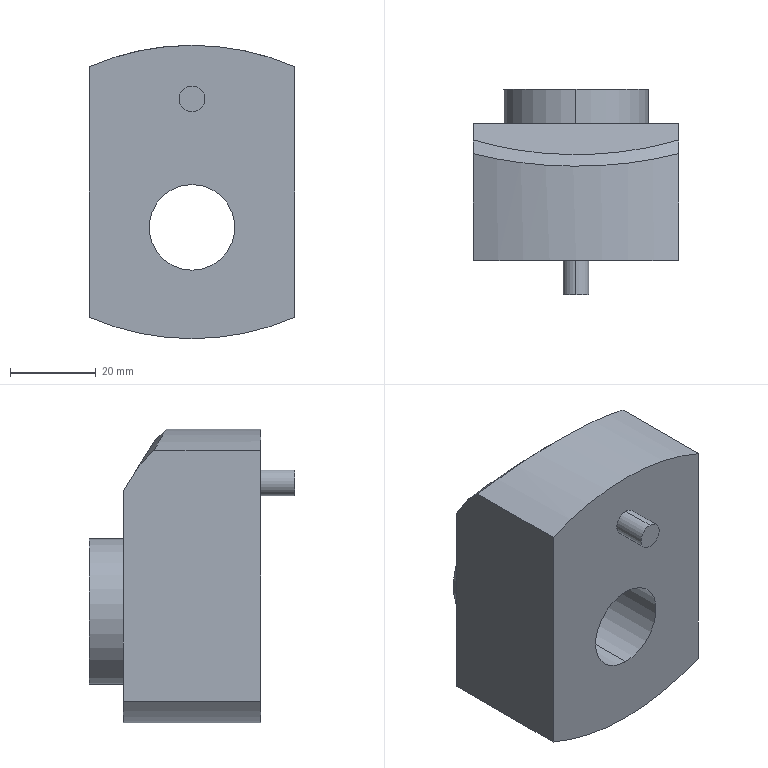Component | SolidWorks | DigitalDisplay.0-1 | 1 solid | 17 faces | box 48 x 48 x 68.5 mm | volume 92589 mm3 | cylinder 9 | plane 7 | spline 1 | commonest cylinder face diameters 120.2 x3 6 x2 20 x2 34 x2
STEP:
#1=COLOUR_RGB('',0.7922,0.8196,0.9333);
#2=FILL_AREA_STYLE_COLOUR('',#1);
#3=FILL_AREA_STYLE('',(#2));
#4=SURFACE_STYLE_FILL_AREA(#3);
#5=SURFACE_SIDE_STYLE('',(#4));
#6=SURFACE_STYLE_USAGE(.BOTH.,#5);
#7=PRESENTATION_STYLE_ASSIGNMENT((#6));
#8=CARTESIAN_POINT('',(-1.162,10.299,19.094));
#9=VERTEX_POINT('',#8);
#10=CARTESIAN_POINT('',(-1.162,10.299,19.331));
#11=VERTEX_POINT('',#10);
#12=CARTESIAN_POINT('',(-1.162,10.299,19.213));
#13=DIRECTION('',(0.,-1.,0.));
#14=DIRECTION('',(0.,0.,-1.));
#15=AXIS2_PLACEMENT_3D('',#12,#13,#14);
#16=CIRCLE('',#15,0.1181);
#17=EDGE_CURVE('',#9,#11,#16,.T.);
#18=ORIENTED_EDGE('',*,*,#17,.F.);
#19=CARTESIAN_POINT('',(-1.162,10.614,19.094));
#20=VERTEX_POINT('',#19);
#21=CARTESIAN_POINT('',(-1.162,10.299,19.094));
#22=DIRECTION('',(0.,1.,0.));
#23=VECTOR('',#22,39.37);
#24=LINE('',#21,#23);
#25=EDGE_CURVE('',#9,#20,#24,.T.);
#26=ORIENTED_EDGE('',*,*,#25,.T.);
#27=CARTESIAN_POINT('',(-1.162,10.614,19.331));
#28=VERTEX_POINT('',#27);
#29=CARTESIAN_POINT('',(-1.162,10.614,19.213));
#30=DIRECTION('',(0.,-1.,0.));
#31=DIRECTION('',(0.,0.,-1.));
#32=AXIS2_PLACEMENT_3D('',#29,#30,#31);
#33=CIRCLE('',#32,0.1181);
#34=EDGE_CURVE('',#20,#28,#33,.T.);
#35=ORIENTED_EDGE('',*,*,#34,.T.);
#36=CARTESIAN_POINT('',(-1.162,10.299,19.331));
#37=DIRECTION('',(0.,1.,0.));
#38=VECTOR('',#37,39.37);
#39=LINE('',#36,#38);
#40=EDGE_CURVE('',#11,#28,#39,.T.);
#41=ORIENTED_EDGE('',*,*,#40,.F.);
#42=EDGE_LOOP('',(#18,#26,#35,#41));
#43=FACE_OUTER_BOUND('',#42,.T.);
#44=CARTESIAN_POINT('',(-1.162,10.299,19.213));
#45=DIRECTION('',(0.,1.,0.));
#46=DIRECTION('',(0.,0.,1.));
#47=AXIS2_PLACEMENT_3D('',#44,#45,#46);
#48=CYLINDRICAL_SURFACE('',#47,0.1181);
#49=ADVANCED_FACE('',(#43),#48,.T.);
#50=CARTESIAN_POINT('',(-1.162,10.614,17.638));
#51=VERTEX_POINT('',#50);
#52=CARTESIAN_POINT('',(-1.162,10.614,18.425));
#53=VERTEX_POINT('',#52);
#54=CARTESIAN_POINT('',(-1.162,10.614,18.031));
#55=DIRECTION('',(0.,1.,0.));
#56=DIRECTION('',(0.,0.,1.));
#57=AXIS2_PLACEMENT_3D('',#54,#55,#56);
#58=CIRCLE('',#57,0.3937);
#59=EDGE_CURVE('',#51,#53,#58,.T.);
#60=ORIENTED_EDGE('',*,*,#59,.F.);
#61=CARTESIAN_POINT('',(-1.162,12.189,17.638));
#62=VERTEX_POINT('',#61);
#63=CARTESIAN_POINT('',(-1.162,10.614,17.638));
#64=DIRECTION('',(0.,1.,0.));
#65=VECTOR('',#64,39.37);
#66=LINE('',#63,#65);
#67=EDGE_CURVE('',#51,#62,#66,.T.);
#68=ORIENTED_EDGE('',*,*,#67,.T.);
#69=CARTESIAN_POINT('',(-1.162,12.189,18.425));
#70=VERTEX_POINT('',#69);
#71=CARTESIAN_POINT('',(-1.162,12.189,18.031));
#72=DIRECTION('',(0.,1.,0.));
#73=DIRECTION('',(0.,0.,1.));
#74=AXIS2_PLACEMENT_3D('',#71,#72,#73);
#75=CIRCLE('',#74,0.3937);
#76=EDGE_CURVE('',#62,#70,#75,.T.);
#77=ORIENTED_EDGE('',*,*,#76,.T.);
#78=CARTESIAN_POINT('',(-1.162,10.614,18.425));
#79=DIRECTION('',(0.,1.,0.));
#80=VECTOR('',#79,39.37);
#81=LINE('',#78,#80);
#82=EDGE_CURVE('',#53,#70,#81,.T.);
#83=ORIENTED_EDGE('',*,*,#82,.F.);
#84=EDGE_LOOP('',(#60,#68,#77,#83));
#85=FACE_OUTER_BOUND('',#84,.T.);
#86=CARTESIAN_POINT('',(-1.162,10.614,18.031));
#87=DIRECTION('',(0.,1.,0.));
#88=DIRECTION('',(0.,0.,1.));
#89=AXIS2_PLACEMENT_3D('',#86,#87,#88);
#90=CYLINDRICAL_SURFACE('',#89,0.3937);
#91=ADVANCED_FACE('',(#85),#90,.F.);
#92=CARTESIAN_POINT('',(-1.162,12.189,18.701));
#93=VERTEX_POINT('',#92);
#94=CARTESIAN_POINT('',(-1.162,12.189,17.362));
#95=VERTEX_POINT('',#94);
#96=CARTESIAN_POINT('',(-1.162,12.189,18.031));
#97=DIRECTION('',(0.,1.,0.));
#98=DIRECTION('',(0.,0.,1.));
#99=AXIS2_PLACEMENT_3D('',#96,#97,#98);
#100=CIRCLE('',#99,0.6693);
#101=EDGE_CURVE('',#93,#95,#100,.T.);
#102=ORIENTED_EDGE('',*,*,#101,.F.);
#103=CARTESIAN_POINT('',(-1.162,11.874,18.701));
#104=VERTEX_POINT('',#103);
#105=CARTESIAN_POINT('',(-1.162,12.189,18.701));
#106=DIRECTION('',(0.,-1.,0.));
#107=VECTOR('',#106,39.37);
#108=LINE('',#105,#107);
#109=EDGE_CURVE('',#93,#104,#108,.T.);
#110=ORIENTED_EDGE('',*,*,#109,.T.);
#111=CARTESIAN_POINT('',(-1.162,11.874,17.362));
#112=VERTEX_POINT('',#111);
#113=CARTESIAN_POINT('',(-1.162,11.874,18.031));
#114=DIRECTION('',(0.,1.,0.));
#115=DIRECTION('',(0.,0.,-1.));
#116=AXIS2_PLACEMENT_3D('',#113,#114,#115);
#117=CIRCLE('',#116,0.6693);
#118=EDGE_CURVE('',#104,#112,#117,.T.);
#119=ORIENTED_EDGE('',*,*,#118,.T.);
#120=CARTESIAN_POINT('',(-1.162,12.189,17.362));
#121=DIRECTION('',(0.,-1.,0.));
#122=VECTOR('',#121,39.37);
#123=LINE('',#120,#122);
#124=EDGE_CURVE('',#95,#112,#123,.T.);
#125=ORIENTED_EDGE('',*,*,#124,.F.);
#126=EDGE_LOOP('',(#102,#110,#119,#125));
#127=FACE_OUTER_BOUND('',#126,.T.);
#128=CARTESIAN_POINT('',(-1.162,12.189,18.031));
#129=DIRECTION('',(0.,-1.,0.));
#130=DIRECTION('',(0.,0.,-1.));
#131=AXIS2_PLACEMENT_3D('',#128,#129,#130);
#132=CYLINDRICAL_SURFACE('',#131,0.6693);
#133=ADVANCED_FACE('',(#127),#132,.T.);
#134=CARTESIAN_POINT('',(-1.162,11.874,17.008));
#135=VERTEX_POINT('',#134);
#136=CARTESIAN_POINT('',(-2.107,11.874,17.205));
#137=VERTEX_POINT('',#136);
#138=CARTESIAN_POINT('',(-1.162,11.874,19.374));
#139=DIRECTION('',(0.,1.,0.));
#140=DIRECTION('',(0.,0.,-1.));
#141=AXIS2_PLACEMENT_3D('',#138,#139,#140);
#142=CIRCLE('',#141,2.366);
#143=EDGE_CURVE('',#135,#137,#142,.T.);
#144=ORIENTED_EDGE('',*,*,#143,.F.);
#145=CARTESIAN_POINT('',(-1.162,10.614,17.008));
#146=VERTEX_POINT('',#145);
#147=CARTESIAN_POINT('',(-1.162,11.874,17.008));
#148=DIRECTION('',(0.,-1.,0.));
#149=VECTOR('',#148,39.37);
#150=LINE('',#147,#149);
#151=EDGE_CURVE('',#135,#146,#150,.T.);
#152=ORIENTED_EDGE('',*,*,#151,.T.);
#153=CARTESIAN_POINT('',(-2.107,10.614,17.205));
#154=VERTEX_POINT('',#153);
#155=CARTESIAN_POINT('',(-1.162,10.614,19.374));
#156=DIRECTION('',(0.,1.,0.));
#157=DIRECTION('',(0.,0.,-1.));
#158=AXIS2_PLACEMENT_3D('',#155,#156,#157);
#159=CIRCLE('',#158,2.366);
#160=EDGE_CURVE('',#146,#154,#159,.T.);
#161=ORIENTED_EDGE('',*,*,#160,.T.);
#162=CARTESIAN_POINT('',(-2.107,11.874,17.205));
#163=DIRECTION('',(0.,-1.,0.));
#164=VECTOR('',#163,39.37);
#165=LINE('',#162,#164);
#166=EDGE_CURVE('',#137,#154,#165,.T.);
#167=ORIENTED_EDGE('',*,*,#166,.F.);
#168=EDGE_LOOP('',(#144,#152,#161,#167));
#169=FACE_OUTER_BOUND('',#168,.T.);
#170=CARTESIAN_POINT('',(-1.162,11.874,19.374));
#171=DIRECTION('',(0.,-1.,0.));
#172=DIRECTION('',(0.,0.,-1.));
#173=AXIS2_PLACEMENT_3D('',#170,#171,#172);
#174=CYLINDRICAL_SURFACE('',#173,2.366);
#175=ADVANCED_FACE('',(#169),#174,.T.);
#176=CARTESIAN_POINT('',(-2.107,11.595,19.508));
#177=VERTEX_POINT('',#176);
#178=CARTESIAN_POINT('',(-2.107,10.614,19.508));
#179=VERTEX_POINT('',#178);
#180=CARTESIAN_POINT('',(-2.107,11.874,19.508));
#181=DIRECTION('',(0.,-1.,0.));
#182=VECTOR('',#181,39.37);
#183=LINE('',#180,#182);
#184=EDGE_CURVE('',#177,#179,#183,.T.);
#185=ORIENTED_EDGE('',*,*,#184,.F.);
#186=CARTESIAN_POINT('',(-2.107,11.722,19.384));
#187=VERTEX_POINT('',#186);
#188=CARTESIAN_POINT('',(-2.107,11.595,19.508));
#189=CARTESIAN_POINT('',(-2.107,11.64,19.464));
#190=CARTESIAN_POINT('',(-2.107,11.682,19.423));
#191=CARTESIAN_POINT('',(-2.107,11.722,19.384));
#192=B_SPLINE_CURVE_WITH_KNOTS('',3,(#188,#189,#190,#191),.UNSPECIFIED.,.F.,.F.,(4,4),(0.,1.),.UNSPECIFIED.);
#193=EDGE_CURVE('',#177,#187,#192,.T.);
#194=ORIENTED_EDGE('',*,*,#193,.T.);
#195=CARTESIAN_POINT('',(-2.107,11.874,19.144));
#196=VERTEX_POINT('',#195);
#197=CARTESIAN_POINT('',(-2.107,12.749,17.758));
#198=DIRECTION('',(0.,-0.534,0.8455));
#199=VECTOR('',#198,39.37);
#200=LINE('',#197,#199);
#201=EDGE_CURVE('',#196,#187,#200,.T.);
#202=ORIENTED_EDGE('',*,*,#201,.F.);
#203=CARTESIAN_POINT('',(-2.107,11.874,17.205));
#204=DIRECTION('',(0.,0.,1.));
#205=VECTOR('',#204,39.37);
#206=LINE('',#203,#205);
#207=EDGE_CURVE('',#137,#196,#206,.T.);
#208=ORIENTED_EDGE('',*,*,#207,.F.);
#209=ORIENTED_EDGE('',*,*,#166,.T.);
#210=CARTESIAN_POINT('',(-2.107,10.614,17.205));
#211=DIRECTION('',(0.,0.,1.));
#212=VECTOR('',#211,39.37);
#213=LINE('',#210,#212);
#214=EDGE_CURVE('',#154,#179,#213,.T.);
#215=ORIENTED_EDGE('',*,*,#214,.T.);
#216=EDGE_LOOP('',(#185,#194,#202,#208,#209,#215));
#217=FACE_OUTER_BOUND('',#216,.T.);
#218=CARTESIAN_POINT('',(-2.107,11.874,17.205));
#219=DIRECTION('',(1.,0.,-0.));
#220=DIRECTION('',(-0.,0.,-1.));
#221=AXIS2_PLACEMENT_3D('',#218,#219,#220);
#222=PLANE('',#221);
#223=ADVANCED_FACE('',(#217),#222,.F.);
#224=CARTESIAN_POINT('',(-0.2168,11.595,19.508));
#225=VERTEX_POINT('',#224);
#226=CARTESIAN_POINT('',(-0.2168,10.614,19.508));
#227=VERTEX_POINT('',#226);
#228=CARTESIAN_POINT('',(-0.2168,11.874,19.508));
#229=DIRECTION('',(0.,-1.,0.));
#230=VECTOR('',#229,39.37);
#231=LINE('',#228,#230);
#232=EDGE_CURVE('',#225,#227,#231,.T.);
#233=ORIENTED_EDGE('',*,*,#232,.F.);
#234=CARTESIAN_POINT('',(-0.2168,11.595,19.508));
#235=CARTESIAN_POINT('',(-0.2542,11.586,19.524));
#236=CARTESIAN_POINT('',(-0.2918,11.577,19.539));
#237=CARTESIAN_POINT('',(-0.3487,11.564,19.561));
#238=CARTESIAN_POINT('',(-0.3772,11.558,19.571));
#239=CARTESIAN_POINT('',(-0.4106,11.551,19.582));
#240=CARTESIAN_POINT('',(-0.425,11.549,19.587));
#241=CARTESIAN_POINT('',(-0.4346,11.547,19.59));
#242=CARTESIAN_POINT('',(-0.4393,11.546,19.592));
#243=CARTESIAN_POINT('',(-0.4829,11.538,19.606));
#244=CARTESIAN_POINT('',(-0.5219,11.531,19.617));
#245=CARTESIAN_POINT('',(-0.5807,11.522,19.632));
#246=CARTESIAN_POINT('',(-0.6101,11.518,19.64));
#247=CARTESIAN_POINT('',(-0.6397,11.514,19.646));
#248=CARTESIAN_POINT('',(-0.6594,11.511,19.651));
#249=CARTESIAN_POINT('',(-0.6691,11.51,19.653));
#250=CARTESIAN_POINT('',(-0.7189,11.504,19.663));
#251=CARTESIAN_POINT('',(-0.7588,11.5,19.671));
#252=CARTESIAN_POINT('',(-0.8188,11.494,19.68));
#253=CARTESIAN_POINT('',(-0.8388,11.493,19.683));
#254=CARTESIAN_POINT('',(-0.8789,11.49,19.688));
#255=CARTESIAN_POINT('',(-0.8989,11.488,19.69));
#256=CARTESIAN_POINT('',(-0.9998,11.482,19.701));
#257=CARTESIAN_POINT('',(-1.081,11.48,19.705));
#258=CARTESIAN_POINT('',(-1.202,11.48,19.705));
#259=CARTESIAN_POINT('',(-1.243,11.48,19.704));
#260=CARTESIAN_POINT('',(-1.303,11.482,19.701));
#261=CARTESIAN_POINT('',(-1.323,11.483,19.699));
#262=CARTESIAN_POINT('',(-1.364,11.485,19.696));
#263=CARTESIAN_POINT('',(-1.384,11.486,19.694));
#264=CARTESIAN_POINT('',(-1.444,11.49,19.688));
#265=CARTESIAN_POINT('',(-1.485,11.493,19.683));
#266=CARTESIAN_POINT('',(-1.545,11.498,19.674));
#267=CARTESIAN_POINT('',(-1.575,11.501,19.669));
#268=CARTESIAN_POINT('',(-1.604,11.504,19.663));
#269=CARTESIAN_POINT('',(-1.624,11.507,19.659));
#270=CARTESIAN_POINT('',(-1.634,11.508,19.657));
#271=CARTESIAN_POINT('',(-1.684,11.514,19.647));
#272=CARTESIAN_POINT('',(-1.723,11.519,19.638));
#273=CARTESIAN_POINT('',(-1.782,11.528,19.622));
#274=CARTESIAN_POINT('',(-1.811,11.533,19.614));
#275=CARTESIAN_POINT('',(-1.845,11.539,19.604));
#276=CARTESIAN_POINT('',(-1.86,11.541,19.599));
#277=CARTESIAN_POINT('',(-1.869,11.543,19.596));
#278=CARTESIAN_POINT('',(-1.874,11.544,19.595));
#279=CARTESIAN_POINT('',(-1.956,11.559,19.569));
#280=CARTESIAN_POINT('',(-2.032,11.576,19.54));
#281=CARTESIAN_POINT('',(-2.107,11.595,19.508));
#282=B_SPLINE_CURVE_WITH_KNOTS('',3,(#234,#235,#236,#237,#238,#239,#240,#241,#242,#243,#244,#245,#246,#247,#248,#249,#250,#251,#252,#253,#254,#255,#256,#257,#258,#259,#260,#261,#262,#263,#264,#265,#266,#267,#268,#269,#270,#271,#272,#273,#274,#275,#276,#277,#278,#279,#280,#281),.UNSPECIFIED.,.F.,.F.,(4,2,1,1,2,2,2,1,2,2,2,2,2,2,2,2,2,2,1,2,2,2,1,1,2,2,4),(0.,0.0625,0.09375,0.1094,0.1172,0.125,0.1875,0.2188,0.2344,0.25,0.3125,0.3438,0.375,0.5,0.5625,0.5938,0.625,0.6875,0.7188,0.7344,0.75,0.8125,0.8438,0.8594,0.8672,0.875,1.),.UNSPECIFIED.);
#283=EDGE_CURVE('',#225,#177,#282,.T.);
#284=ORIENTED_EDGE('',*,*,#283,.T.);
#285=ORIENTED_EDGE('',*,*,#184,.T.);
#286=CARTESIAN_POINT('',(-1.162,10.614,17.339));
#287=DIRECTION('',(0.,1.,0.));
#288=DIRECTION('',(0.,0.,-1.));
#289=AXIS2_PLACEMENT_3D('',#286,#287,#288);
#290=CIRCLE('',#289,2.366);
#291=EDGE_CURVE('',#179,#227,#290,.T.);
#292=ORIENTED_EDGE('',*,*,#291,.T.);
#293=EDGE_LOOP('',(#233,#284,#285,#292));
#294=FACE_OUTER_BOUND('',#293,.T.);
#295=CARTESIAN_POINT('',(-1.162,11.874,17.339));
#296=DIRECTION('',(0.,-1.,0.));
#297=DIRECTION('',(0.,0.,-1.));
#298=AXIS2_PLACEMENT_3D('',#295,#296,#297);
#299=CYLINDRICAL_SURFACE('',#298,2.366);
#300=ADVANCED_FACE('',(#294),#299,.T.);
#301=CARTESIAN_POINT('',(-0.2168,11.722,19.384));
#302=VERTEX_POINT('',#301);
#303=CARTESIAN_POINT('',(-0.2168,11.874,19.144));
#304=VERTEX_POINT('',#303);
#305=CARTESIAN_POINT('',(-0.2168,12.749,17.758));
#306=DIRECTION('',(-0.,0.534,-0.8455));
#307=VECTOR('',#306,39.37);
#308=LINE('',#305,#307);
#309=EDGE_CURVE('',#302,#304,#308,.T.);
#310=ORIENTED_EDGE('',*,*,#309,.F.);
#311=CARTESIAN_POINT('',(-0.2168,11.722,19.384));
#312=CARTESIAN_POINT('',(-0.2168,11.682,19.423));
#313=CARTESIAN_POINT('',(-0.2168,11.64,19.464));
#314=CARTESIAN_POINT('',(-0.2168,11.595,19.508));
#315=B_SPLINE_CURVE_WITH_KNOTS('',3,(#311,#312,#313,#314),.UNSPECIFIED.,.F.,.F.,(4,4),(0.,1.),.UNSPECIFIED.);
#316=EDGE_CURVE('',#302,#225,#315,.T.);
#317=ORIENTED_EDGE('',*,*,#316,.T.);
#318=ORIENTED_EDGE('',*,*,#232,.T.);
#319=CARTESIAN_POINT('',(-0.2168,10.614,17.205));
#320=VERTEX_POINT('',#319);
#321=CARTESIAN_POINT('',(-0.2168,10.614,17.205));
#322=DIRECTION('',(-0.,0.,-1.));
#323=VECTOR('',#322,39.37);
#324=LINE('',#321,#323);
#325=EDGE_CURVE('',#227,#320,#324,.T.);
#326=ORIENTED_EDGE('',*,*,#325,.T.);
#327=CARTESIAN_POINT('',(-0.2168,11.874,17.205));
#328=VERTEX_POINT('',#327);
#329=CARTESIAN_POINT('',(-0.2168,11.874,17.205));
#330=DIRECTION('',(0.,-1.,0.));
#331=VECTOR('',#330,39.37);
#332=LINE('',#329,#331);
#333=EDGE_CURVE('',#328,#320,#332,.T.);
#334=ORIENTED_EDGE('',*,*,#333,.F.);
#335=CARTESIAN_POINT('',(-0.2168,11.874,17.205));
#336=DIRECTION('',(-0.,0.,-1.));
#337=VECTOR('',#336,39.37);
#338=LINE('',#335,#337);
#339=EDGE_CURVE('',#304,#328,#338,.T.);
#340=ORIENTED_EDGE('',*,*,#339,.F.);
#341=EDGE_LOOP('',(#310,#317,#318,#326,#334,#340));
#342=FACE_OUTER_BOUND('',#341,.T.);
#343=CARTESIAN_POINT('',(-0.2168,11.874,17.205));
#344=DIRECTION('',(-1.,0.,0.));
#345=DIRECTION('',(0.,0.,1.));
#346=AXIS2_PLACEMENT_3D('',#343,#344,#345);
#347=PLANE('',#346);
#348=ADVANCED_FACE('',(#342),#347,.F.);
#349=CARTESIAN_POINT('',(-1.162,11.874,18.031));
#350=DIRECTION('',(0.,1.,0.));
#351=DIRECTION('',(0.,0.,-1.));
#352=AXIS2_PLACEMENT_3D('',#349,#350,#351);
#353=CIRCLE('',#352,0.6693);
#354=EDGE_CURVE('',#112,#104,#353,.T.);
#355=ORIENTED_EDGE('',*,*,#354,.F.);
#356=ORIENTED_EDGE('',*,*,#118,.F.);
#357=EDGE_LOOP('',(#355,#356));
#358=FACE_BOUND('',#357,.T.);
#359=CARTESIAN_POINT('',(-1.162,11.874,19.144));
#360=DIRECTION('',(-1.,0.,0.));
#361=VECTOR('',#360,39.37);
#362=LINE('',#359,#361);
#363=EDGE_CURVE('',#304,#196,#362,.T.);
#364=ORIENTED_EDGE('',*,*,#363,.F.);
#365=ORIENTED_EDGE('',*,*,#339,.T.);
#366=CARTESIAN_POINT('',(-1.162,11.874,19.374));
#367=DIRECTION('',(0.,1.,0.));
#368=DIRECTION('',(0.,0.,-1.));
#369=AXIS2_PLACEMENT_3D('',#366,#367,#368);
#370=CIRCLE('',#369,2.366);
#371=EDGE_CURVE('',#328,#135,#370,.T.);
#372=ORIENTED_EDGE('',*,*,#371,.T.);
#373=ORIENTED_EDGE('',*,*,#143,.T.);
#374=ORIENTED_EDGE('',*,*,#207,.T.);
#375=EDGE_LOOP('',(#364,#365,#372,#373,#374));
#376=FACE_OUTER_BOUND('',#375,.T.);
#377=CARTESIAN_POINT('',(-1.162,11.874,19.374));
#378=DIRECTION('',(0.,-1.,0.));
#379=DIRECTION('',(0.,0.,-1.));
#380=AXIS2_PLACEMENT_3D('',#377,#378,#379);
#381=PLANE('',#380);
#382=ADVANCED_FACE('',(#358,#376),#381,.F.);
#383=ORIENTED_EDGE('',*,*,#151,.F.);
#384=ORIENTED_EDGE('',*,*,#371,.F.);
#385=ORIENTED_EDGE('',*,*,#333,.T.);
#386=CARTESIAN_POINT('',(-1.162,10.614,19.374));
#387=DIRECTION('',(0.,1.,0.));
#388=DIRECTION('',(0.,0.,-1.));
#389=AXIS2_PLACEMENT_3D('',#386,#387,#388);
#390=CIRCLE('',#389,2.366);
#391=EDGE_CURVE('',#320,#146,#390,.T.);
#392=ORIENTED_EDGE('',*,*,#391,.T.);
#393=EDGE_LOOP('',(#383,#384,#385,#392));
#394=FACE_OUTER_BOUND('',#393,.T.);
#395=CARTESIAN_POINT('',(-1.162,11.874,19.374));
#396=DIRECTION('',(0.,-1.,0.));
#397=DIRECTION('',(0.,0.,-1.));
#398=AXIS2_PLACEMENT_3D('',#395,#396,#397);
#399=CYLINDRICAL_SURFACE('',#398,2.366);
#400=ADVANCED_FACE('',(#394),#399,.T.);
#401=CARTESIAN_POINT('',(-1.162,10.614,19.213));
#402=DIRECTION('',(0.,-1.,0.));
#403=DIRECTION('',(0.,0.,-1.));
#404=AXIS2_PLACEMENT_3D('',#401,#402,#403);
#405=CIRCLE('',#404,0.1181);
#406=EDGE_CURVE('',#28,#20,#405,.T.);
#407=ORIENTED_EDGE('',*,*,#406,.F.);
#408=ORIENTED_EDGE('',*,*,#34,.F.);
#409=EDGE_LOOP('',(#407,#408));
#410=FACE_BOUND('',#409,.T.);
#411=CARTESIAN_POINT('',(-1.162,10.614,18.031));
#412=DIRECTION('',(0.,1.,0.));
#413=DIRECTION('',(0.,0.,1.));
#414=AXIS2_PLACEMENT_3D('',#411,#412,#413);
#415=CIRCLE('',#414,0.3937);
#416=EDGE_CURVE('',#53,#51,#415,.T.);
#417=ORIENTED_EDGE('',*,*,#416,.T.);
#418=ORIENTED_EDGE('',*,*,#59,.T.);
#419=EDGE_LOOP('',(#417,#418));
#420=FACE_BOUND('',#419,.T.);
#421=ORIENTED_EDGE('',*,*,#391,.F.);
#422=ORIENTED_EDGE('',*,*,#325,.F.);
#423=ORIENTED_EDGE('',*,*,#291,.F.);
#424=ORIENTED_EDGE('',*,*,#214,.F.);
#425=ORIENTED_EDGE('',*,*,#160,.F.);
#426=EDGE_LOOP('',(#421,#422,#423,#424,#425));
#427=FACE_OUTER_BOUND('',#426,.T.);
#428=CARTESIAN_POINT('',(-1.162,10.614,19.374));
#429=DIRECTION('',(0.,-1.,0.));
#430=DIRECTION('',(0.,0.,-1.));
#431=AXIS2_PLACEMENT_3D('',#428,#429,#430);
#432=PLANE('',#431);
#433=ADVANCED_FACE('',(#410,#420,#427),#432,.T.);
#434=ORIENTED_EDGE('',*,*,#109,.F.);
#435=CARTESIAN_POINT('',(-1.162,12.189,18.031));
#436=DIRECTION('',(0.,1.,0.));
#437=DIRECTION('',(0.,0.,1.));
#438=AXIS2_PLACEMENT_3D('',#435,#436,#437);
#439=CIRCLE('',#438,0.6693);
#440=EDGE_CURVE('',#95,#93,#439,.T.);
#441=ORIENTED_EDGE('',*,*,#440,.F.);
#442=ORIENTED_EDGE('',*,*,#124,.T.);
#443=ORIENTED_EDGE('',*,*,#354,.T.);
#444=EDGE_LOOP('',(#434,#441,#442,#443));
#445=FACE_OUTER_BOUND('',#444,.T.);
#446=CARTESIAN_POINT('',(-1.162,12.189,18.031));
#447=DIRECTION('',(0.,-1.,0.));
#448=DIRECTION('',(0.,0.,-1.));
#449=AXIS2_PLACEMENT_3D('',#446,#447,#448);
#450=CYLINDRICAL_SURFACE('',#449,0.6693);
#451=ADVANCED_FACE('',(#445),#450,.T.);
#452=CARTESIAN_POINT('',(-1.162,12.189,18.031));
#453=DIRECTION('',(0.,1.,0.));
#454=DIRECTION('',(0.,0.,1.));
#455=AXIS2_PLACEMENT_3D('',#452,#453,#454);
#456=CIRCLE('',#455,0.3937);
#457=EDGE_CURVE('',#70,#62,#456,.T.);
#458=ORIENTED_EDGE('',*,*,#457,.F.);
#459=ORIENTED_EDGE('',*,*,#76,.F.);
#460=EDGE_LOOP('',(#458,#459));
#461=FACE_BOUND('',#460,.T.);
#462=ORIENTED_EDGE('',*,*,#440,.T.);
#463=ORIENTED_EDGE('',*,*,#101,.T.);
#464=EDGE_LOOP('',(#462,#463));
#465=FACE_OUTER_BOUND('',#464,.T.);
#466=CARTESIAN_POINT('',(-1.162,12.189,18.031));
#467=DIRECTION('',(0.,1.,0.));
#468=DIRECTION('',(0.,0.,1.));
#469=AXIS2_PLACEMENT_3D('',#466,#467,#468);
#470=PLANE('',#469);
#471=ADVANCED_FACE('',(#461,#465),#470,.T.);
#472=ORIENTED_EDGE('',*,*,#67,.F.);
#473=ORIENTED_EDGE('',*,*,#416,.F.);
#474=ORIENTED_EDGE('',*,*,#82,.T.);
#475=ORIENTED_EDGE('',*,*,#457,.T.);
#476=EDGE_LOOP('',(#472,#473,#474,#475));
#477=FACE_OUTER_BOUND('',#476,.T.);
#478=CARTESIAN_POINT('',(-1.162,10.614,18.031));
#479=DIRECTION('',(0.,1.,0.));
#480=DIRECTION('',(0.,0.,1.));
#481=AXIS2_PLACEMENT_3D('',#478,#479,#480);
#482=CYLINDRICAL_SURFACE('',#481,0.3937);
#483=ADVANCED_FACE('',(#477),#482,.F.);
#484=ORIENTED_EDGE('',*,*,#201,.T.);
#485=CARTESIAN_POINT('',(-2.107,11.722,19.384));
#486=CARTESIAN_POINT('',(-2.033,11.7,19.419));
#487=CARTESIAN_POINT('',(-1.958,11.68,19.45));
#488=CARTESIAN_POINT('',(-1.804,11.646,19.503));
#489=CARTESIAN_POINT('',(-1.726,11.632,19.526));
#490=CARTESIAN_POINT('',(-1.567,11.61,19.562));
#491=CARTESIAN_POINT('',(-1.486,11.601,19.575));
#492=CARTESIAN_POINT('',(-1.324,11.59,19.593));
#493=CARTESIAN_POINT('',(-1.243,11.587,19.598));
#494=CARTESIAN_POINT('',(-1.08,11.587,19.598));
#495=CARTESIAN_POINT('',(-0.9989,11.59,19.593));
#496=CARTESIAN_POINT('',(-0.837,11.601,19.575));
#497=CARTESIAN_POINT('',(-0.7567,11.61,19.562));
#498=CARTESIAN_POINT('',(-0.5978,11.632,19.526));
#499=CARTESIAN_POINT('',(-0.5195,11.646,19.503));
#500=CARTESIAN_POINT('',(-0.3656,11.68,19.45));
#501=CARTESIAN_POINT('',(-0.2903,11.7,19.419));
#502=CARTESIAN_POINT('',(-0.2168,11.722,19.384));
#503=B_SPLINE_CURVE_WITH_KNOTS('',3,(#485,#486,#487,#488,#489,#490,#491,#492,#493,#494,#495,#496,#497,#498,#499,#500,#501,#502),.UNSPECIFIED.,.F.,.F.,(4,2,2,2,2,2,2,2,4),(0.,0.125,0.25,0.375,0.5,0.625,0.75,0.875,1.),.UNSPECIFIED.);
#504=EDGE_CURVE('',#187,#302,#503,.T.);
#505=ORIENTED_EDGE('',*,*,#504,.T.);
#506=ORIENTED_EDGE('',*,*,#309,.T.);
#507=ORIENTED_EDGE('',*,*,#363,.T.);
#508=EDGE_LOOP('',(#484,#505,#506,#507));
#509=FACE_OUTER_BOUND('',#508,.T.);
#510=CARTESIAN_POINT('',(-6.669,11.874,19.144));
#511=DIRECTION('',(0.,0.8455,0.534));
#512=DIRECTION('',(0.,-0.534,0.8455));
#513=AXIS2_PLACEMENT_3D('',#510,#511,#512);
#514=PLANE('',#513);
#515=ADVANCED_FACE('',(#509),#514,.T.);
#516=ORIENTED_EDGE('',*,*,#193,.F.);
#517=ORIENTED_EDGE('',*,*,#283,.F.);
#518=ORIENTED_EDGE('',*,*,#316,.F.);
#519=ORIENTED_EDGE('',*,*,#504,.F.);
#520=EDGE_LOOP('',(#516,#517,#518,#519));
#521=FACE_OUTER_BOUND('',#520,.T.);
#522=CARTESIAN_POINT('',(-2.194,11.75,19.34));
#523=CARTESIAN_POINT('',(-2.115,11.723,19.382));
#524=CARTESIAN_POINT('',(-2.033,11.7,19.419));
#525=CARTESIAN_POINT('',(-1.866,11.659,19.484));
#526=CARTESIAN_POINT('',(-1.78,11.642,19.511));
#527=CARTESIAN_POINT('',(-1.607,11.614,19.554));
#528=CARTESIAN_POINT('',(-1.519,11.604,19.57));
#529=CARTESIAN_POINT('',(-1.341,11.59,19.592));
#530=CARTESIAN_POINT('',(-1.251,11.587,19.598));
#531=CARTESIAN_POINT('',(-1.072,11.587,19.598));
#532=CARTESIAN_POINT('',(-0.9826,11.59,19.592));
#533=CARTESIAN_POINT('',(-0.8048,11.604,19.57));
#534=CARTESIAN_POINT('',(-0.7166,11.614,19.554));
#535=CARTESIAN_POINT('',(-0.5429,11.642,19.511));
#536=CARTESIAN_POINT('',(-0.4573,11.659,19.484));
#537=CARTESIAN_POINT('',(-0.2902,11.7,19.419));
#538=CARTESIAN_POINT('',(-0.2086,11.723,19.382));
#539=CARTESIAN_POINT('',(-0.1296,11.75,19.34));
#540=CARTESIAN_POINT('',(-2.276,11.643,19.426));
#541=CARTESIAN_POINT('',(-2.191,11.616,19.472));
#542=CARTESIAN_POINT('',(-2.102,11.593,19.512));
#543=CARTESIAN_POINT('',(-1.922,11.552,19.581));
#544=CARTESIAN_POINT('',(-1.83,11.535,19.611));
#545=CARTESIAN_POINT('',(-1.642,11.508,19.657));
#546=CARTESIAN_POINT('',(-1.547,11.497,19.675));
#547=CARTESIAN_POINT('',(-1.355,11.483,19.699));
#548=CARTESIAN_POINT('',(-1.258,11.48,19.705));
#549=CARTESIAN_POINT('',(-1.065,11.48,19.705));
#550=CARTESIAN_POINT('',(-0.9683,11.483,19.699));
#551=CARTESIAN_POINT('',(-0.7764,11.497,19.675));
#552=CARTESIAN_POINT('',(-0.6812,11.508,19.657));
#553=CARTESIAN_POINT('',(-0.4936,11.535,19.611));
#554=CARTESIAN_POINT('',(-0.4013,11.552,19.581));
#555=CARTESIAN_POINT('',(-0.2209,11.593,19.512));
#556=CARTESIAN_POINT('',(-0.1328,11.616,19.472));
#557=CARTESIAN_POINT('',(-0.04752,11.643,19.426));
#558=B_SPLINE_SURFACE_WITH_KNOTS('',1,3,((#522,#523,#524,#525,#526,#527,#528,#529,#530,#531,#532,#533,#534,#535,#536,#537,#538,#539),(#540,#541,#542,#543,#544,#545,#546,#547,#548,#549,#550,#551,#552,#553,#554,#555,#556,#557)),.UNSPECIFIED.,.F.,.F.,.F.,(2,2),(4,2,2,2,2,2,2,2,4),(0.,1.),(5.793,5.915,6.038,6.161,6.283,6.406,6.528,6.651,6.773),.UNSPECIFIED.);
#559=ADVANCED_FACE('',(#521),#558,.T.);
#560=ORIENTED_EDGE('',*,*,#25,.F.);
#561=CARTESIAN_POINT('',(-1.162,10.299,19.213));
#562=DIRECTION('',(0.,-1.,0.));
#563=DIRECTION('',(0.,0.,-1.));
#564=AXIS2_PLACEMENT_3D('',#561,#562,#563);
#565=CIRCLE('',#564,0.1181);
#566=EDGE_CURVE('',#11,#9,#565,.T.);
#567=ORIENTED_EDGE('',*,*,#566,.F.);
#568=ORIENTED_EDGE('',*,*,#40,.T.);
#569=ORIENTED_EDGE('',*,*,#406,.T.);
#570=EDGE_LOOP('',(#560,#567,#568,#569));
#571=FACE_OUTER_BOUND('',#570,.T.);
#572=CARTESIAN_POINT('',(-1.162,10.299,19.213));
#573=DIRECTION('',(0.,1.,0.));
#574=DIRECTION('',(0.,0.,1.));
#575=AXIS2_PLACEMENT_3D('',#572,#573,#574);
#576=CYLINDRICAL_SURFACE('',#575,0.1181);
#577=ADVANCED_FACE('',(#571),#576,.T.);
#578=ORIENTED_EDGE('',*,*,#566,.T.);
#579=ORIENTED_EDGE('',*,*,#17,.T.);
#580=EDGE_LOOP('',(#578,#579));
#581=FACE_OUTER_BOUND('',#580,.T.);
#582=CARTESIAN_POINT('',(-1.162,10.299,19.213));
#583=DIRECTION('',(0.,-1.,0.));
#584=DIRECTION('',(0.,0.,-1.));
#585=AXIS2_PLACEMENT_3D('',#582,#583,#584);
#586=PLANE('',#585);
#587=ADVANCED_FACE('',(#581),#586,.T.);
#588=CLOSED_SHELL('',(#49,#91,#133,#175,#223,#300,#348,#382,#400,#433,#451,#471,#483,#515,#559,#577,#587));
#589=MANIFOLD_SOLID_BREP('',#588);
#590=STYLED_ITEM('',(#7),#589);
#591=PRESENTATION_LAYER_ASSIGNMENT('','',(#590));
#592=CARTESIAN_POINT('',(0.,0.,0.));
#593=DIRECTION('',(0.,0.,1.));
#594=DIRECTION('',(1.,0.,0.));
#595=AXIS2_PLACEMENT_3D('',#592,#593,#594);
#596=(LENGTH_UNIT()NAMED_UNIT(*)SI_UNIT($,.METRE.));
#597=LENGTH_MEASURE_WITH_UNIT(LENGTH_MEASURE(0.0254),#596);
#598=DIMENSIONAL_EXPONENTS(1.,0.,0.,0.,0.,0.,0.);
#599=(CONVERSION_BASED_UNIT('',#597)LENGTH_UNIT()NAMED_UNIT(#598));
#600=UNCERTAINTY_MEASURE_WITH_UNIT(LENGTH_MEASURE(0.00001),#599,'','');
#601=(NAMED_UNIT(*)PLANE_ANGLE_UNIT()SI_UNIT($,.RADIAN.));
#602=(NAMED_UNIT(*)SI_UNIT($,.STERADIAN.)SOLID_ANGLE_UNIT());
#603=(GEOMETRIC_REPRESENTATION_CONTEXT(3)GLOBAL_UNCERTAINTY_ASSIGNED_CONTEXT((#600))GLOBAL_UNIT_ASSIGNED_CONTEXT((#599,#601,#602))REPRESENTATION_CONTEXT('',''));
#604=ADVANCED_BREP_SHAPE_REPRESENTATION('',(#589,#595),#603);
#605=(LENGTH_UNIT()NAMED_UNIT(*)SI_UNIT($,.METRE.));
#606=LENGTH_MEASURE_WITH_UNIT(LENGTH_MEASURE(0.0254),#605);
#607=DIMENSIONAL_EXPONENTS(1.,0.,0.,0.,0.,0.,0.);
#608=(CONVERSION_BASED_UNIT('',#606)LENGTH_UNIT()NAMED_UNIT(#607));
#609=UNCERTAINTY_MEASURE_WITH_UNIT(LENGTH_MEASURE(0.00001),#608,'','');
#610=(NAMED_UNIT(*)PLANE_ANGLE_UNIT()SI_UNIT($,.RADIAN.));
#611=(NAMED_UNIT(*)SI_UNIT($,.STERADIAN.)SOLID_ANGLE_UNIT());
#612=(GEOMETRIC_REPRESENTATION_CONTEXT(3)GLOBAL_UNCERTAINTY_ASSIGNED_CONTEXT((#609))GLOBAL_UNIT_ASSIGNED_CONTEXT((#608,#610,#611))REPRESENTATION_CONTEXT('',''));
#613=MECHANICAL_DESIGN_GEOMETRIC_PRESENTATION_REPRESENTATION('',(#590),#612);